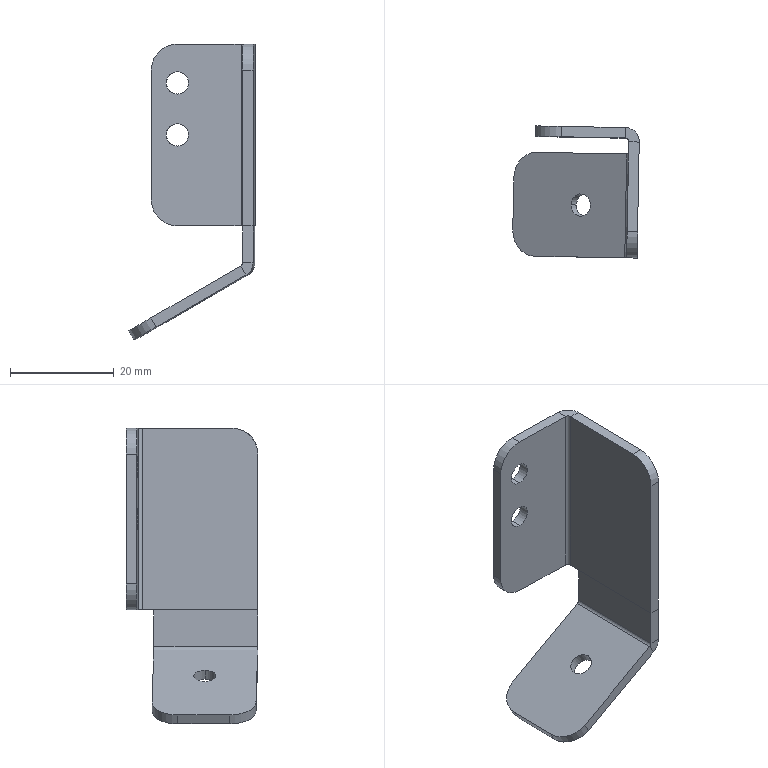Component | SolidWorks | DM17A08-02-004-1 | 2 solids | 39 faces | box 24.34 x 25.37 x 56.96 mm | volume 4173 mm3 | plane 24 | cylinder 15 | commonest cylinder face diameters 4.3 x6 10 x5 5.473 x2 1.473 x2
STEP:
#1=COLOUR_RGB('',0.7922,0.8196,0.9333);
#2=FILL_AREA_STYLE_COLOUR('',#1);
#3=FILL_AREA_STYLE('',(#2));
#4=SURFACE_STYLE_FILL_AREA(#3);
#5=SURFACE_SIDE_STYLE('',(#4));
#6=SURFACE_STYLE_USAGE(.BOTH.,#5);
#7=PRESENTATION_STYLE_ASSIGNMENT((#6));
#8=CARTESIAN_POINT('',(17.975,18.731,37.871));
#9=VERTEX_POINT('',#8);
#10=CARTESIAN_POINT('',(17.975,18.731,38.04));
#11=VERTEX_POINT('',#10);
#12=CARTESIAN_POINT('',(17.975,18.731,37.956));
#13=DIRECTION('',(0.01873,0.9998,-0.));
#14=DIRECTION('',(0.,0.,1.));
#15=AXIS2_PLACEMENT_3D('',#12,#13,#14);
#16=CIRCLE('',#15,0.08465);
#17=EDGE_CURVE('',#9,#11,#16,.T.);
#18=ORIENTED_EDGE('',*,*,#17,.F.);
#19=CARTESIAN_POINT('',(17.977,18.81,37.871));
#20=VERTEX_POINT('',#19);
#21=CARTESIAN_POINT('',(17.977,18.81,37.871));
#22=DIRECTION('',(0.01873,0.9998,-0.));
#23=VECTOR('',#22,39.37);
#24=LINE('',#21,#23);
#25=EDGE_CURVE('',#9,#20,#24,.T.);
#26=ORIENTED_EDGE('',*,*,#25,.T.);
#27=CARTESIAN_POINT('',(17.977,18.81,38.04));
#28=VERTEX_POINT('',#27);
#29=CARTESIAN_POINT('',(17.977,18.81,37.956));
#30=DIRECTION('',(0.01873,0.9998,-0.));
#31=DIRECTION('',(0.,0.,1.));
#32=AXIS2_PLACEMENT_3D('',#29,#30,#31);
#33=CIRCLE('',#32,0.08465);
#34=EDGE_CURVE('',#20,#28,#33,.T.);
#35=ORIENTED_EDGE('',*,*,#34,.T.);
#36=CARTESIAN_POINT('',(17.977,18.81,38.04));
#37=DIRECTION('',(0.01873,0.9998,-0.));
#38=VECTOR('',#37,39.37);
#39=LINE('',#36,#38);
#40=EDGE_CURVE('',#11,#28,#39,.T.);
#41=ORIENTED_EDGE('',*,*,#40,.F.);
#42=EDGE_LOOP('',(#18,#26,#35,#41));
#43=FACE_OUTER_BOUND('',#42,.T.);
#44=CARTESIAN_POINT('',(17.977,18.81,37.956));
#45=DIRECTION('',(0.01873,0.9998,-0.));
#46=DIRECTION('',(0.,0.,1.));
#47=AXIS2_PLACEMENT_3D('',#44,#45,#46);
#48=CYLINDRICAL_SURFACE('',#47,0.08465);
#49=ADVANCED_FACE('',(#43),#48,.F.);
#50=CARTESIAN_POINT('',(17.975,18.731,37.477));
#51=VERTEX_POINT('',#50);
#52=CARTESIAN_POINT('',(17.975,18.731,37.646));
#53=VERTEX_POINT('',#52);
#54=CARTESIAN_POINT('',(17.975,18.731,37.562));
#55=DIRECTION('',(0.01873,0.9998,-0.));
#56=DIRECTION('',(0.,0.,1.));
#57=AXIS2_PLACEMENT_3D('',#54,#55,#56);
#58=CIRCLE('',#57,0.08465);
#59=EDGE_CURVE('',#51,#53,#58,.T.);
#60=ORIENTED_EDGE('',*,*,#59,.F.);
#61=CARTESIAN_POINT('',(17.977,18.81,37.477));
#62=VERTEX_POINT('',#61);
#63=CARTESIAN_POINT('',(17.977,18.81,37.477));
#64=DIRECTION('',(0.01873,0.9998,-0.));
#65=VECTOR('',#64,39.37);
#66=LINE('',#63,#65);
#67=EDGE_CURVE('',#51,#62,#66,.T.);
#68=ORIENTED_EDGE('',*,*,#67,.T.);
#69=CARTESIAN_POINT('',(17.977,18.81,37.646));
#70=VERTEX_POINT('',#69);
#71=CARTESIAN_POINT('',(17.977,18.81,37.562));
#72=DIRECTION('',(0.01873,0.9998,-0.));
#73=DIRECTION('',(0.,0.,1.));
#74=AXIS2_PLACEMENT_3D('',#71,#72,#73);
#75=CIRCLE('',#74,0.08465);
#76=EDGE_CURVE('',#62,#70,#75,.T.);
#77=ORIENTED_EDGE('',*,*,#76,.T.);
#78=CARTESIAN_POINT('',(17.977,18.81,37.646));
#79=DIRECTION('',(0.01873,0.9998,-0.));
#80=VECTOR('',#79,39.37);
#81=LINE('',#78,#80);
#82=EDGE_CURVE('',#53,#70,#81,.T.);
#83=ORIENTED_EDGE('',*,*,#82,.F.);
#84=EDGE_LOOP('',(#60,#68,#77,#83));
#85=FACE_OUTER_BOUND('',#84,.T.);
#86=CARTESIAN_POINT('',(17.977,18.81,37.562));
#87=DIRECTION('',(0.01873,0.9998,-0.));
#88=DIRECTION('',(0.,0.,1.));
#89=AXIS2_PLACEMENT_3D('',#86,#87,#88);
#90=CYLINDRICAL_SURFACE('',#89,0.08465);
#91=ADVANCED_FACE('',(#85),#90,.F.);
#92=CARTESIAN_POINT('',(18.565,18.691,38.251));
#93=VERTEX_POINT('',#92);
#94=CARTESIAN_POINT('',(18.486,18.692,38.251));
#95=VERTEX_POINT('',#94);
#96=CARTESIAN_POINT('',(18.565,18.691,38.251));
#97=DIRECTION('',(-0.9998,0.01873,-0.));
#98=VECTOR('',#97,39.37);
#99=LINE('',#96,#98);
#100=EDGE_CURVE('',#93,#95,#99,.T.);
#101=ORIENTED_EDGE('',*,*,#100,.F.);
#102=CARTESIAN_POINT('',(18.459,18.801,38.251));
#103=VERTEX_POINT('',#102);
#104=CARTESIAN_POINT('',(18.457,18.693,38.251));
#105=DIRECTION('',(-0.,-0.,-1.));
#106=DIRECTION('',(0.9998,-0.01873,0.));
#107=AXIS2_PLACEMENT_3D('',#104,#105,#106);
#108=CIRCLE('',#107,0.1077);
#109=EDGE_CURVE('',#103,#93,#108,.T.);
#110=ORIENTED_EDGE('',*,*,#109,.F.);
#111=CARTESIAN_POINT('',(18.458,18.722,38.251));
#112=VERTEX_POINT('',#111);
#113=CARTESIAN_POINT('',(18.458,18.722,38.251));
#114=DIRECTION('',(0.01873,0.9998,-0.));
#115=VECTOR('',#114,39.37);
#116=LINE('',#113,#115);
#117=EDGE_CURVE('',#112,#103,#116,.T.);
#118=ORIENTED_EDGE('',*,*,#117,.F.);
#119=CARTESIAN_POINT('',(18.457,18.693,38.251));
#120=DIRECTION('',(-0.,-0.,-1.));
#121=DIRECTION('',(0.9998,-0.01873,0.));
#122=AXIS2_PLACEMENT_3D('',#119,#120,#121);
#123=CIRCLE('',#122,0.029);
#124=EDGE_CURVE('',#112,#95,#123,.T.);
#125=ORIENTED_EDGE('',*,*,#124,.T.);
#126=EDGE_LOOP('',(#101,#110,#118,#125));
#127=FACE_OUTER_BOUND('',#126,.T.);
#128=CARTESIAN_POINT('',(18.565,18.691,38.251));
#129=DIRECTION('',(0.,0.,1.));
#130=DIRECTION('',(0.9998,-0.01873,0.));
#131=AXIS2_PLACEMENT_3D('',#128,#129,#130);
#132=PLANE('',#131);
#133=ADVANCED_FACE('',(#127),#132,.T.);
#134=CARTESIAN_POINT('',(18.474,18.013,38.251));
#135=VERTEX_POINT('',#134);
#136=CARTESIAN_POINT('',(18.488,18.8,38.251));
#137=DIRECTION('',(-0.01873,-0.9998,0.));
#138=VECTOR('',#137,39.37);
#139=LINE('',#136,#138);
#140=EDGE_CURVE('',#95,#135,#139,.T.);
#141=ORIENTED_EDGE('',*,*,#140,.T.);
#142=CARTESIAN_POINT('',(18.552,18.011,38.251));
#143=VERTEX_POINT('',#142);
#144=CARTESIAN_POINT('',(18.445,18.013,38.251));
#145=DIRECTION('',(0.9998,-0.01873,0.));
#146=VECTOR('',#145,39.37);
#147=LINE('',#144,#146);
#148=EDGE_CURVE('',#135,#143,#147,.T.);
#149=ORIENTED_EDGE('',*,*,#148,.T.);
#150=CARTESIAN_POINT('',(18.567,18.799,38.251));
#151=DIRECTION('',(-0.01873,-0.9998,0.));
#152=VECTOR('',#151,39.37);
#153=LINE('',#150,#152);
#154=EDGE_CURVE('',#93,#143,#153,.T.);
#155=ORIENTED_EDGE('',*,*,#154,.F.);
#156=ORIENTED_EDGE('',*,*,#100,.T.);
#157=EDGE_LOOP('',(#141,#149,#155,#156));
#158=FACE_OUTER_BOUND('',#157,.T.);
#159=CARTESIAN_POINT('',(18.458,18.722,38.251));
#160=DIRECTION('',(0.,0.,1.));
#161=DIRECTION('',(0.9998,-0.01873,0.));
#162=AXIS2_PLACEMENT_3D('',#159,#160,#161);
#163=PLANE('',#162);
#164=ADVANCED_FACE('',(#158),#163,.T.);
#165=CARTESIAN_POINT('',(18.459,18.801,36.873));
#166=VERTEX_POINT('',#165);
#167=CARTESIAN_POINT('',(18.458,18.722,36.873));
#168=VERTEX_POINT('',#167);
#169=CARTESIAN_POINT('',(18.459,18.801,36.873));
#170=DIRECTION('',(-0.01873,-0.9998,0.));
#171=VECTOR('',#170,39.37);
#172=LINE('',#169,#171);
#173=EDGE_CURVE('',#166,#168,#172,.T.);
#174=ORIENTED_EDGE('',*,*,#173,.F.);
#175=CARTESIAN_POINT('',(18.565,18.691,36.873));
#176=VERTEX_POINT('',#175);
#177=CARTESIAN_POINT('',(18.457,18.693,36.873));
#178=DIRECTION('',(-0.,-0.,-1.));
#179=DIRECTION('',(0.9998,-0.01873,0.));
#180=AXIS2_PLACEMENT_3D('',#177,#178,#179);
#181=CIRCLE('',#180,0.1077);
#182=EDGE_CURVE('',#166,#176,#181,.T.);
#183=ORIENTED_EDGE('',*,*,#182,.T.);
#184=CARTESIAN_POINT('',(18.486,18.692,36.873));
#185=VERTEX_POINT('',#184);
#186=CARTESIAN_POINT('',(18.486,18.692,36.873));
#187=DIRECTION('',(0.9998,-0.01873,0.));
#188=VECTOR('',#187,39.37);
#189=LINE('',#186,#188);
#190=EDGE_CURVE('',#185,#176,#189,.T.);
#191=ORIENTED_EDGE('',*,*,#190,.F.);
#192=CARTESIAN_POINT('',(18.457,18.693,36.873));
#193=DIRECTION('',(-0.,-0.,-1.));
#194=DIRECTION('',(0.9998,-0.01873,0.));
#195=AXIS2_PLACEMENT_3D('',#192,#193,#194);
#196=CIRCLE('',#195,0.029);
#197=EDGE_CURVE('',#168,#185,#196,.T.);
#198=ORIENTED_EDGE('',*,*,#197,.F.);
#199=EDGE_LOOP('',(#174,#183,#191,#198));
#200=FACE_OUTER_BOUND('',#199,.T.);
#201=CARTESIAN_POINT('',(18.459,18.801,36.873));
#202=DIRECTION('',(-0.,-0.,-1.));
#203=DIRECTION('',(-0.9998,0.01873,-0.));
#204=AXIS2_PLACEMENT_3D('',#201,#202,#203);
#205=PLANE('',#204);
#206=ADVANCED_FACE('',(#200),#205,.T.);
#207=CARTESIAN_POINT('',(17.975,18.731,36.873));
#208=VERTEX_POINT('',#207);
#209=CARTESIAN_POINT('',(17.778,18.735,36.873));
#210=DIRECTION('',(0.9998,-0.01873,0.));
#211=VECTOR('',#210,39.37);
#212=LINE('',#209,#211);
#213=EDGE_CURVE('',#208,#168,#212,.T.);
#214=ORIENTED_EDGE('',*,*,#213,.F.);
#215=CARTESIAN_POINT('',(17.977,18.81,36.873));
#216=VERTEX_POINT('',#215);
#217=CARTESIAN_POINT('',(17.975,18.702,36.873));
#218=DIRECTION('',(0.01873,0.9998,-0.));
#219=VECTOR('',#218,39.37);
#220=LINE('',#217,#219);
#221=EDGE_CURVE('',#208,#216,#220,.T.);
#222=ORIENTED_EDGE('',*,*,#221,.T.);
#223=CARTESIAN_POINT('',(17.78,18.813,36.873));
#224=DIRECTION('',(0.9998,-0.01873,0.));
#225=VECTOR('',#224,39.37);
#226=LINE('',#223,#225);
#227=EDGE_CURVE('',#216,#166,#226,.T.);
#228=ORIENTED_EDGE('',*,*,#227,.T.);
#229=ORIENTED_EDGE('',*,*,#173,.T.);
#230=EDGE_LOOP('',(#214,#222,#228,#229));
#231=FACE_OUTER_BOUND('',#230,.T.);
#232=CARTESIAN_POINT('',(18.486,18.692,36.873));
#233=DIRECTION('',(-0.,-0.,-1.));
#234=DIRECTION('',(-0.9998,0.01873,-0.));
#235=AXIS2_PLACEMENT_3D('',#232,#233,#234);
#236=PLANE('',#235);
#237=ADVANCED_FACE('',(#231),#236,.T.);
#238=CARTESIAN_POINT('',(18.47,17.816,38.054));
#239=VERTEX_POINT('',#238);
#240=CARTESIAN_POINT('',(18.47,17.816,36.873));
#241=VERTEX_POINT('',#240);
#242=CARTESIAN_POINT('',(18.47,17.816,38.251));
#243=DIRECTION('',(-0.,-0.,-1.));
#244=VECTOR('',#243,39.37);
#245=LINE('',#242,#244);
#246=EDGE_CURVE('',#239,#241,#245,.T.);
#247=ORIENTED_EDGE('',*,*,#246,.F.);
#248=CARTESIAN_POINT('',(18.474,18.013,38.054));
#249=DIRECTION('',(-0.9998,0.01873,-0.));
#250=DIRECTION('',(0.01873,0.9998,0.));
#251=AXIS2_PLACEMENT_3D('',#248,#249,#250);
#252=CIRCLE('',#251,0.1969);
#253=EDGE_CURVE('',#239,#135,#252,.T.);
#254=ORIENTED_EDGE('',*,*,#253,.T.);
#255=ORIENTED_EDGE('',*,*,#140,.F.);
#256=CARTESIAN_POINT('',(18.486,18.692,38.251));
#257=DIRECTION('',(-0.,-0.,-1.));
#258=VECTOR('',#257,39.37);
#259=LINE('',#256,#258);
#260=EDGE_CURVE('',#95,#185,#259,.T.);
#261=ORIENTED_EDGE('',*,*,#260,.T.);
#262=CARTESIAN_POINT('',(18.488,18.8,36.873));
#263=DIRECTION('',(-0.01873,-0.9998,0.));
#264=VECTOR('',#263,39.37);
#265=LINE('',#262,#264);
#266=EDGE_CURVE('',#185,#241,#265,.T.);
#267=ORIENTED_EDGE('',*,*,#266,.T.);
#268=EDGE_LOOP('',(#247,#254,#255,#261,#267));
#269=FACE_OUTER_BOUND('',#268,.T.);
#270=CARTESIAN_POINT('',(18.488,18.8,38.251));
#271=DIRECTION('',(0.9998,-0.01873,0.));
#272=DIRECTION('',(0.01873,0.9998,-0.));
#273=AXIS2_PLACEMENT_3D('',#270,#271,#272);
#274=PLANE('',#273);
#275=ADVANCED_FACE('',(#269),#274,.F.);
#276=CARTESIAN_POINT('',(18.549,17.815,38.054));
#277=VERTEX_POINT('',#276);
#278=CARTESIAN_POINT('',(18.549,17.815,36.873));
#279=VERTEX_POINT('',#278);
#280=CARTESIAN_POINT('',(18.549,17.815,38.251));
#281=DIRECTION('',(-0.,-0.,-1.));
#282=VECTOR('',#281,39.37);
#283=LINE('',#280,#282);
#284=EDGE_CURVE('',#277,#279,#283,.T.);
#285=ORIENTED_EDGE('',*,*,#284,.F.);
#286=CARTESIAN_POINT('',(18.549,17.815,38.054));
#287=DIRECTION('',(-0.9998,0.01873,-0.));
#288=VECTOR('',#287,39.37);
#289=LINE('',#286,#288);
#290=EDGE_CURVE('',#277,#239,#289,.T.);
#291=ORIENTED_EDGE('',*,*,#290,.T.);
#292=ORIENTED_EDGE('',*,*,#246,.T.);
#293=CARTESIAN_POINT('',(18.549,17.815,36.873));
#294=DIRECTION('',(-0.9998,0.01873,-0.));
#295=VECTOR('',#294,39.37);
#296=LINE('',#293,#295);
#297=EDGE_CURVE('',#279,#241,#296,.T.);
#298=ORIENTED_EDGE('',*,*,#297,.F.);
#299=EDGE_LOOP('',(#285,#291,#292,#298));
#300=FACE_OUTER_BOUND('',#299,.T.);
#301=CARTESIAN_POINT('',(18.549,17.815,38.251));
#302=DIRECTION('',(-0.01873,-0.9998,0.));
#303=DIRECTION('',(-0.,-0.,-1.));
#304=AXIS2_PLACEMENT_3D('',#301,#302,#303);
#305=PLANE('',#304);
#306=ADVANCED_FACE('',(#300),#305,.T.);
#307=ORIENTED_EDGE('',*,*,#154,.T.);
#308=CARTESIAN_POINT('',(18.552,18.011,38.054));
#309=DIRECTION('',(0.9998,-0.01873,0.));
#310=DIRECTION('',(0.01873,0.9998,0.));
#311=AXIS2_PLACEMENT_3D('',#308,#309,#310);
#312=CIRCLE('',#311,0.1969);
#313=EDGE_CURVE('',#143,#277,#312,.T.);
#314=ORIENTED_EDGE('',*,*,#313,.T.);
#315=ORIENTED_EDGE('',*,*,#284,.T.);
#316=CARTESIAN_POINT('',(18.567,18.799,36.873));
#317=DIRECTION('',(-0.01873,-0.9998,0.));
#318=VECTOR('',#317,39.37);
#319=LINE('',#316,#318);
#320=EDGE_CURVE('',#176,#279,#319,.T.);
#321=ORIENTED_EDGE('',*,*,#320,.F.);
#322=CARTESIAN_POINT('',(18.565,18.691,38.251));
#323=DIRECTION('',(-0.,-0.,-1.));
#324=VECTOR('',#323,39.37);
#325=LINE('',#322,#324);
#326=EDGE_CURVE('',#93,#176,#325,.T.);
#327=ORIENTED_EDGE('',*,*,#326,.F.);
#328=EDGE_LOOP('',(#307,#314,#315,#321,#327));
#329=FACE_OUTER_BOUND('',#328,.T.);
#330=CARTESIAN_POINT('',(18.567,18.799,38.251));
#331=DIRECTION('',(0.9998,-0.01873,0.));
#332=DIRECTION('',(0.01873,0.9998,-0.));
#333=AXIS2_PLACEMENT_3D('',#330,#331,#332);
#334=PLANE('',#333);
#335=ADVANCED_FACE('',(#329),#334,.T.);
#336=ORIENTED_EDGE('',*,*,#182,.F.);
#337=CARTESIAN_POINT('',(18.459,18.801,38.251));
#338=DIRECTION('',(-0.,-0.,-1.));
#339=VECTOR('',#338,39.37);
#340=LINE('',#337,#339);
#341=EDGE_CURVE('',#103,#166,#340,.T.);
#342=ORIENTED_EDGE('',*,*,#341,.F.);
#343=ORIENTED_EDGE('',*,*,#109,.T.);
#344=ORIENTED_EDGE('',*,*,#326,.T.);
#345=EDGE_LOOP('',(#336,#342,#343,#344));
#346=FACE_OUTER_BOUND('',#345,.T.);
#347=CARTESIAN_POINT('',(18.457,18.693,38.251));
#348=DIRECTION('',(-0.,-0.,-1.));
#349=DIRECTION('',(-0.9998,0.01873,0.));
#350=AXIS2_PLACEMENT_3D('',#347,#348,#349);
#351=CYLINDRICAL_SURFACE('',#350,0.1077);
#352=ADVANCED_FACE('',(#346),#351,.T.);
#353=CARTESIAN_POINT('',(17.977,18.81,37.956));
#354=DIRECTION('',(0.01873,0.9998,-0.));
#355=DIRECTION('',(0.,0.,1.));
#356=AXIS2_PLACEMENT_3D('',#353,#354,#355);
#357=CIRCLE('',#356,0.08465);
#358=EDGE_CURVE('',#28,#20,#357,.T.);
#359=ORIENTED_EDGE('',*,*,#358,.F.);
#360=ORIENTED_EDGE('',*,*,#34,.F.);
#361=EDGE_LOOP('',(#359,#360));
#362=FACE_BOUND('',#361,.T.);
#363=CARTESIAN_POINT('',(17.977,18.81,37.562));
#364=DIRECTION('',(0.01873,0.9998,-0.));
#365=DIRECTION('',(0.,0.,1.));
#366=AXIS2_PLACEMENT_3D('',#363,#364,#365);
#367=CIRCLE('',#366,0.08465);
#368=EDGE_CURVE('',#70,#62,#367,.T.);
#369=ORIENTED_EDGE('',*,*,#368,.F.);
#370=ORIENTED_EDGE('',*,*,#76,.F.);
#371=EDGE_LOOP('',(#369,#370));
#372=FACE_BOUND('',#371,.T.);
#373=ORIENTED_EDGE('',*,*,#227,.F.);
#374=CARTESIAN_POINT('',(17.78,18.813,37.069));
#375=VERTEX_POINT('',#374);
#376=CARTESIAN_POINT('',(17.977,18.81,37.069));
#377=DIRECTION('',(0.01873,0.9998,-0.));
#378=DIRECTION('',(0.,0.,1.));
#379=AXIS2_PLACEMENT_3D('',#376,#377,#378);
#380=CIRCLE('',#379,0.1969);
#381=EDGE_CURVE('',#216,#375,#380,.T.);
#382=ORIENTED_EDGE('',*,*,#381,.T.);
#383=CARTESIAN_POINT('',(17.78,18.813,38.054));
#384=VERTEX_POINT('',#383);
#385=CARTESIAN_POINT('',(17.78,18.813,38.251));
#386=DIRECTION('',(-0.,-0.,-1.));
#387=VECTOR('',#386,39.37);
#388=LINE('',#385,#387);
#389=EDGE_CURVE('',#384,#375,#388,.T.);
#390=ORIENTED_EDGE('',*,*,#389,.F.);
#391=CARTESIAN_POINT('',(17.977,18.81,38.251));
#392=VERTEX_POINT('',#391);
#393=CARTESIAN_POINT('',(17.977,18.81,38.054));
#394=DIRECTION('',(0.01873,0.9998,-0.));
#395=DIRECTION('',(0.,0.,1.));
#396=AXIS2_PLACEMENT_3D('',#393,#394,#395);
#397=CIRCLE('',#396,0.1969);
#398=EDGE_CURVE('',#384,#392,#397,.T.);
#399=ORIENTED_EDGE('',*,*,#398,.T.);
#400=CARTESIAN_POINT('',(17.78,18.813,38.251));
#401=DIRECTION('',(0.9998,-0.01873,0.));
#402=VECTOR('',#401,39.37);
#403=LINE('',#400,#402);
#404=EDGE_CURVE('',#392,#103,#403,.T.);
#405=ORIENTED_EDGE('',*,*,#404,.T.);
#406=ORIENTED_EDGE('',*,*,#341,.T.);
#407=EDGE_LOOP('',(#373,#382,#390,#399,#405,#406));
#408=FACE_OUTER_BOUND('',#407,.T.);
#409=CARTESIAN_POINT('',(17.78,18.813,38.251));
#410=DIRECTION('',(0.01873,0.9998,-0.));
#411=DIRECTION('',(0.,0.,1.));
#412=AXIS2_PLACEMENT_3D('',#409,#410,#411);
#413=PLANE('',#412);
#414=ADVANCED_FACE('',(#362,#372,#408),#413,.T.);
#415=ORIENTED_EDGE('',*,*,#389,.T.);
#416=CARTESIAN_POINT('',(17.778,18.735,37.069));
#417=VERTEX_POINT('',#416);
#418=CARTESIAN_POINT('',(17.778,18.735,37.069));
#419=DIRECTION('',(-0.01873,-0.9998,0.));
#420=VECTOR('',#419,39.37);
#421=LINE('',#418,#420);
#422=EDGE_CURVE('',#375,#417,#421,.T.);
#423=ORIENTED_EDGE('',*,*,#422,.T.);
#424=CARTESIAN_POINT('',(17.778,18.735,38.054));
#425=VERTEX_POINT('',#424);
#426=CARTESIAN_POINT('',(17.778,18.735,38.251));
#427=DIRECTION('',(-0.,-0.,-1.));
#428=VECTOR('',#427,39.37);
#429=LINE('',#426,#428);
#430=EDGE_CURVE('',#425,#417,#429,.T.);
#431=ORIENTED_EDGE('',*,*,#430,.F.);
#432=CARTESIAN_POINT('',(17.778,18.735,38.054));
#433=DIRECTION('',(0.01873,0.9998,-0.));
#434=VECTOR('',#433,39.37);
#435=LINE('',#432,#434);
#436=EDGE_CURVE('',#425,#384,#435,.T.);
#437=ORIENTED_EDGE('',*,*,#436,.T.);
#438=EDGE_LOOP('',(#415,#423,#431,#437));
#439=FACE_OUTER_BOUND('',#438,.T.);
#440=CARTESIAN_POINT('',(17.778,18.735,38.251));
#441=DIRECTION('',(-0.9998,0.01873,-0.));
#442=DIRECTION('',(0.,0.,1.));
#443=AXIS2_PLACEMENT_3D('',#440,#441,#442);
#444=PLANE('',#443);
#445=ADVANCED_FACE('',(#439),#444,.T.);
#446=CARTESIAN_POINT('',(17.975,18.731,37.956));
#447=DIRECTION('',(0.01873,0.9998,-0.));
#448=DIRECTION('',(0.,0.,1.));
#449=AXIS2_PLACEMENT_3D('',#446,#447,#448);
#450=CIRCLE('',#449,0.08465);
#451=EDGE_CURVE('',#11,#9,#450,.T.);
#452=ORIENTED_EDGE('',*,*,#451,.T.);
#453=ORIENTED_EDGE('',*,*,#17,.T.);
#454=EDGE_LOOP('',(#452,#453));
#455=FACE_BOUND('',#454,.T.);
#456=CARTESIAN_POINT('',(17.975,18.731,37.562));
#457=DIRECTION('',(0.01873,0.9998,-0.));
#458=DIRECTION('',(0.,0.,1.));
#459=AXIS2_PLACEMENT_3D('',#456,#457,#458);
#460=CIRCLE('',#459,0.08465);
#461=EDGE_CURVE('',#53,#51,#460,.T.);
#462=ORIENTED_EDGE('',*,*,#461,.T.);
#463=ORIENTED_EDGE('',*,*,#59,.T.);
#464=EDGE_LOOP('',(#462,#463));
#465=FACE_BOUND('',#464,.T.);
#466=ORIENTED_EDGE('',*,*,#430,.T.);
#467=CARTESIAN_POINT('',(17.975,18.731,37.069));
#468=DIRECTION('',(-0.01873,-0.9998,0.));
#469=DIRECTION('',(0.,0.,1.));
#470=AXIS2_PLACEMENT_3D('',#467,#468,#469);
#471=CIRCLE('',#470,0.1969);
#472=EDGE_CURVE('',#417,#208,#471,.T.);
#473=ORIENTED_EDGE('',*,*,#472,.T.);
#474=ORIENTED_EDGE('',*,*,#213,.T.);
#475=CARTESIAN_POINT('',(18.458,18.722,38.251));
#476=DIRECTION('',(-0.,-0.,-1.));
#477=VECTOR('',#476,39.37);
#478=LINE('',#475,#477);
#479=EDGE_CURVE('',#112,#168,#478,.T.);
#480=ORIENTED_EDGE('',*,*,#479,.F.);
#481=CARTESIAN_POINT('',(17.975,18.731,38.251));
#482=VERTEX_POINT('',#481);
#483=CARTESIAN_POINT('',(17.778,18.735,38.251));
#484=DIRECTION('',(0.9998,-0.01873,0.));
#485=VECTOR('',#484,39.37);
#486=LINE('',#483,#485);
#487=EDGE_CURVE('',#482,#112,#486,.T.);
#488=ORIENTED_EDGE('',*,*,#487,.F.);
#489=CARTESIAN_POINT('',(17.975,18.731,38.054));
#490=DIRECTION('',(-0.01873,-0.9998,0.));
#491=DIRECTION('',(0.,0.,1.));
#492=AXIS2_PLACEMENT_3D('',#489,#490,#491);
#493=CIRCLE('',#492,0.1969);
#494=EDGE_CURVE('',#482,#425,#493,.T.);
#495=ORIENTED_EDGE('',*,*,#494,.T.);
#496=EDGE_LOOP('',(#466,#473,#474,#480,#488,#495));
#497=FACE_OUTER_BOUND('',#496,.T.);
#498=CARTESIAN_POINT('',(17.778,18.735,38.251));
#499=DIRECTION('',(0.01873,0.9998,-0.));
#500=DIRECTION('',(0.,0.,1.));
#501=AXIS2_PLACEMENT_3D('',#498,#499,#500);
#502=PLANE('',#501);
#503=ADVANCED_FACE('',(#455,#465,#497),#502,.F.);
#504=ORIENTED_EDGE('',*,*,#197,.T.);
#505=ORIENTED_EDGE('',*,*,#260,.F.);
#506=ORIENTED_EDGE('',*,*,#124,.F.);
#507=ORIENTED_EDGE('',*,*,#479,.T.);
#508=EDGE_LOOP('',(#504,#505,#506,#507));
#509=FACE_OUTER_BOUND('',#508,.T.);
#510=CARTESIAN_POINT('',(18.457,18.693,38.251));
#511=DIRECTION('',(-0.,-0.,-1.));
#512=DIRECTION('',(-0.9998,0.01873,0.));
#513=AXIS2_PLACEMENT_3D('',#510,#511,#512);
#514=CYLINDRICAL_SURFACE('',#513,0.029);
#515=ADVANCED_FACE('',(#509),#514,.F.);
#516=ORIENTED_EDGE('',*,*,#404,.F.);
#517=CARTESIAN_POINT('',(17.975,18.702,38.251));
#518=DIRECTION('',(-0.01873,-0.9998,0.));
#519=VECTOR('',#518,39.37);
#520=LINE('',#517,#519);
#521=EDGE_CURVE('',#392,#482,#520,.T.);
#522=ORIENTED_EDGE('',*,*,#521,.T.);
#523=ORIENTED_EDGE('',*,*,#487,.T.);
#524=ORIENTED_EDGE('',*,*,#117,.T.);
#525=EDGE_LOOP('',(#516,#522,#523,#524));
#526=FACE_OUTER_BOUND('',#525,.T.);
#527=CARTESIAN_POINT('',(18.457,18.693,38.251));
#528=DIRECTION('',(0.,0.,1.));
#529=DIRECTION('',(0.9998,-0.01873,0.));
#530=AXIS2_PLACEMENT_3D('',#527,#528,#529);
#531=PLANE('',#530);
#532=ADVANCED_FACE('',(#526),#531,.T.);
#533=ORIENTED_EDGE('',*,*,#266,.F.);
#534=ORIENTED_EDGE('',*,*,#190,.T.);
#535=ORIENTED_EDGE('',*,*,#320,.T.);
#536=ORIENTED_EDGE('',*,*,#297,.T.);
#537=EDGE_LOOP('',(#533,#534,#535,#536));
#538=FACE_OUTER_BOUND('',#537,.T.);
#539=CARTESIAN_POINT('',(18.457,18.693,36.873));
#540=DIRECTION('',(0.,0.,1.));
#541=DIRECTION('',(0.9998,-0.01873,0.));
#542=AXIS2_PLACEMENT_3D('',#539,#540,#541);
#543=PLANE('',#542);
#544=ADVANCED_FACE('',(#538),#543,.F.);
#545=ORIENTED_EDGE('',*,*,#67,.F.);
#546=ORIENTED_EDGE('',*,*,#461,.F.);
#547=ORIENTED_EDGE('',*,*,#82,.T.);
#548=ORIENTED_EDGE('',*,*,#368,.T.);
#549=EDGE_LOOP('',(#545,#546,#547,#548));
#550=FACE_OUTER_BOUND('',#549,.T.);
#551=CARTESIAN_POINT('',(17.977,18.81,37.562));
#552=DIRECTION('',(0.01873,0.9998,-0.));
#553=DIRECTION('',(0.,0.,1.));
#554=AXIS2_PLACEMENT_3D('',#551,#552,#553);
#555=CYLINDRICAL_SURFACE('',#554,0.08465);
#556=ADVANCED_FACE('',(#550),#555,.F.);
#557=ORIENTED_EDGE('',*,*,#25,.F.);
#558=ORIENTED_EDGE('',*,*,#451,.F.);
#559=ORIENTED_EDGE('',*,*,#40,.T.);
#560=ORIENTED_EDGE('',*,*,#358,.T.);
#561=EDGE_LOOP('',(#557,#558,#559,#560));
#562=FACE_OUTER_BOUND('',#561,.T.);
#563=CARTESIAN_POINT('',(17.977,18.81,37.956));
#564=DIRECTION('',(0.01873,0.9998,-0.));
#565=DIRECTION('',(0.,0.,1.));
#566=AXIS2_PLACEMENT_3D('',#563,#564,#565);
#567=CYLINDRICAL_SURFACE('',#566,0.08465);
#568=ADVANCED_FACE('',(#562),#567,.F.);
#569=ORIENTED_EDGE('',*,*,#472,.F.);
#570=ORIENTED_EDGE('',*,*,#422,.F.);
#571=ORIENTED_EDGE('',*,*,#381,.F.);
#572=ORIENTED_EDGE('',*,*,#221,.F.);
#573=EDGE_LOOP('',(#569,#570,#571,#572));
#574=FACE_OUTER_BOUND('',#573,.T.);
#575=CARTESIAN_POINT('',(17.975,18.702,37.069));
#576=DIRECTION('',(0.01873,0.9998,-0.));
#577=DIRECTION('',(0.,0.,1.));
#578=AXIS2_PLACEMENT_3D('',#575,#576,#577);
#579=CYLINDRICAL_SURFACE('',#578,0.1969);
#580=ADVANCED_FACE('',(#574),#579,.T.);
#581=ORIENTED_EDGE('',*,*,#313,.F.);
#582=ORIENTED_EDGE('',*,*,#148,.F.);
#583=ORIENTED_EDGE('',*,*,#253,.F.);
#584=ORIENTED_EDGE('',*,*,#290,.F.);
#585=EDGE_LOOP('',(#581,#582,#583,#584));
#586=FACE_OUTER_BOUND('',#585,.T.);
#587=CARTESIAN_POINT('',(18.552,18.011,38.054));
#588=DIRECTION('',(-0.9998,0.01873,-0.));
#589=DIRECTION('',(0.,0.,1.));
#590=AXIS2_PLACEMENT_3D('',#587,#588,#589);
#591=CYLINDRICAL_SURFACE('',#590,0.1969);
#592=ADVANCED_FACE('',(#586),#591,.T.);
#593=ORIENTED_EDGE('',*,*,#494,.F.);
#594=ORIENTED_EDGE('',*,*,#521,.F.);
#595=ORIENTED_EDGE('',*,*,#398,.F.);
#596=ORIENTED_EDGE('',*,*,#436,.F.);
#597=EDGE_LOOP('',(#593,#594,#595,#596));
#598=FACE_OUTER_BOUND('',#597,.T.);
#599=CARTESIAN_POINT('',(17.975,18.731,38.054));
#600=DIRECTION('',(0.01873,0.9998,-0.));
#601=DIRECTION('',(0.,0.,1.));
#602=AXIS2_PLACEMENT_3D('',#599,#600,#601);
#603=CYLINDRICAL_SURFACE('',#602,0.1969);
#604=ADVANCED_FACE('',(#598),#603,.T.);
#605=CLOSED_SHELL('',(#49,#91,#133,#164,#206,#237,#275,#306,#335,#352,#414,#445,#503,#515,#532,#544,#556,#568,#580,#592,#604));
#606=MANIFOLD_SOLID_BREP('',#605);
#607=STYLED_ITEM('',(#7),#606);
#608=PRESENTATION_LAYER_ASSIGNMENT('','',(#607));
#609=COLOUR_RGB('',0.7922,0.8196,0.9333);
#610=FILL_AREA_STYLE_COLOUR('',#609);
#611=FILL_AREA_STYLE('',(#610));
#612=SURFACE_STYLE_FILL_AREA(#611);
#613=SURFACE_SIDE_STYLE('',(#612));
#614=SURFACE_STYLE_USAGE(.BOTH.,#613);
#615=PRESENTATION_STYLE_ASSIGNMENT((#614));
#616=CARTESIAN_POINT('',(18.088,18.217,36.261));
#617=VERTEX_POINT('',#616);
#618=CARTESIAN_POINT('',(18.235,18.214,36.346));
#619=VERTEX_POINT('',#618);
#620=CARTESIAN_POINT('',(18.161,18.216,36.303));
#621=DIRECTION('',(-0.4999,0.009366,0.866));
#622=DIRECTION('',(0.8659,-0.01622,0.5));
#623=AXIS2_PLACEMENT_3D('',#620,#621,#622);
#624=CIRCLE('',#623,0.08465);
#625=EDGE_CURVE('',#617,#619,#624,.T.);
#626=ORIENTED_EDGE('',*,*,#625,.F.);
#627=CARTESIAN_POINT('',(18.049,18.218,36.329));
#628=VERTEX_POINT('',#627);
#629=CARTESIAN_POINT('',(18.049,18.218,36.329));
#630=DIRECTION('',(-0.4999,0.009366,0.866));
#631=VECTOR('',#630,39.37);
#632=LINE('',#629,#631);
#633=EDGE_CURVE('',#617,#628,#632,.T.);
#634=ORIENTED_EDGE('',*,*,#633,.T.);
#635=CARTESIAN_POINT('',(18.195,18.215,36.414));
#636=VERTEX_POINT('',#635);
#637=CARTESIAN_POINT('',(18.122,18.216,36.371));
#638=DIRECTION('',(-0.4999,0.009366,0.866));
#639=DIRECTION('',(0.8659,-0.01622,0.5));
#640=AXIS2_PLACEMENT_3D('',#637,#638,#639);
#641=CIRCLE('',#640,0.08465);
#642=EDGE_CURVE('',#628,#636,#641,.T.);
#643=ORIENTED_EDGE('',*,*,#642,.T.);
#644=CARTESIAN_POINT('',(18.195,18.215,36.414));
#645=DIRECTION('',(-0.4999,0.009366,0.866));
#646=VECTOR('',#645,39.37);
#647=LINE('',#644,#646);
#648=EDGE_CURVE('',#619,#636,#647,.T.);
#649=ORIENTED_EDGE('',*,*,#648,.F.);
#650=EDGE_LOOP('',(#626,#634,#643,#649));
#651=FACE_OUTER_BOUND('',#650,.T.);
#652=CARTESIAN_POINT('',(18.122,18.216,36.371));
#653=DIRECTION('',(-0.4999,0.009366,0.866));
#654=DIRECTION('',(0.8659,-0.01622,0.5));
#655=AXIS2_PLACEMENT_3D('',#652,#653,#654);
#656=CYLINDRICAL_SURFACE('',#655,0.08465);
#657=ADVANCED_FACE('',(#651),#656,.F.);
#658=CARTESIAN_POINT('',(18.161,18.216,36.303));
#659=DIRECTION('',(-0.4999,0.009366,0.866));
#660=DIRECTION('',(0.8659,-0.01622,0.5));
#661=AXIS2_PLACEMENT_3D('',#658,#659,#660);
#662=CIRCLE('',#661,0.08465);
#663=EDGE_CURVE('',#619,#617,#662,.T.);
#664=ORIENTED_EDGE('',*,*,#663,.T.);
#665=ORIENTED_EDGE('',*,*,#625,.T.);
#666=EDGE_LOOP('',(#664,#665));
#667=FACE_BOUND('',#666,.T.);
#668=CARTESIAN_POINT('',(17.646,18.028,36.008));
#669=VERTEX_POINT('',#668);
#670=CARTESIAN_POINT('',(17.654,18.422,36.008));
#671=VERTEX_POINT('',#670);
#672=CARTESIAN_POINT('',(17.657,18.619,36.008));
#673=DIRECTION('',(0.01873,0.9998,-0.));
#674=VECTOR('',#673,39.37);
#675=LINE('',#672,#674);
#676=EDGE_CURVE('',#669,#671,#675,.T.);
#677=ORIENTED_EDGE('',*,*,#676,.T.);
#678=CARTESIAN_POINT('',(17.828,18.616,36.106));
#679=VERTEX_POINT('',#678);
#680=CARTESIAN_POINT('',(17.824,18.419,36.106));
#681=DIRECTION('',(0.4999,-0.009366,-0.866));
#682=DIRECTION('',(0.8659,-0.01622,0.5));
#683=AXIS2_PLACEMENT_3D('',#680,#681,#682);
#684=CIRCLE('',#683,0.1969);
#685=EDGE_CURVE('',#671,#679,#684,.T.);
#686=ORIENTED_EDGE('',*,*,#685,.T.);
#687=CARTESIAN_POINT('',(18.509,18.603,36.5));
#688=VERTEX_POINT('',#687);
#689=CARTESIAN_POINT('',(18.813,18.597,36.675));
#690=DIRECTION('',(-0.8659,0.01622,-0.5));
#691=VECTOR('',#690,39.37);
#692=LINE('',#689,#691);
#693=EDGE_CURVE('',#688,#679,#692,.T.);
#694=ORIENTED_EDGE('',*,*,#693,.F.);
#695=CARTESIAN_POINT('',(18.495,17.816,36.5));
#696=VERTEX_POINT('',#695);
#697=CARTESIAN_POINT('',(18.509,18.603,36.5));
#698=DIRECTION('',(0.01873,0.9998,-0.));
#699=VECTOR('',#698,39.37);
#700=LINE('',#697,#699);
#701=EDGE_CURVE('',#696,#688,#700,.T.);
#702=ORIENTED_EDGE('',*,*,#701,.F.);
#703=CARTESIAN_POINT('',(17.813,17.828,36.106));
#704=VERTEX_POINT('',#703);
#705=CARTESIAN_POINT('',(18.798,17.81,36.675));
#706=DIRECTION('',(-0.8659,0.01622,-0.5));
#707=VECTOR('',#706,39.37);
#708=LINE('',#705,#707);
#709=EDGE_CURVE('',#696,#704,#708,.T.);
#710=ORIENTED_EDGE('',*,*,#709,.T.);
#711=CARTESIAN_POINT('',(17.817,18.025,36.106));
#712=DIRECTION('',(0.4999,-0.009366,-0.866));
#713=DIRECTION('',(0.8659,-0.01622,0.5));
#714=AXIS2_PLACEMENT_3D('',#711,#712,#713);
#715=CIRCLE('',#714,0.1969);
#716=EDGE_CURVE('',#704,#669,#715,.T.);
#717=ORIENTED_EDGE('',*,*,#716,.T.);
#718=EDGE_LOOP('',(#677,#686,#694,#702,#710,#717));
#719=FACE_OUTER_BOUND('',#718,.T.);
#720=CARTESIAN_POINT('',(18.813,18.597,36.675));
#721=DIRECTION('',(-0.4999,0.009366,0.866));
#722=DIRECTION('',(0.8659,-0.01622,0.5));
#723=AXIS2_PLACEMENT_3D('',#720,#721,#722);
#724=PLANE('',#723);
#725=ADVANCED_FACE('',(#667,#719),#724,.F.);
#726=CARTESIAN_POINT('',(18.455,17.816,36.568));
#727=VERTEX_POINT('',#726);
#728=CARTESIAN_POINT('',(17.774,17.829,36.175));
#729=VERTEX_POINT('',#728);
#730=CARTESIAN_POINT('',(18.759,17.811,36.744));
#731=DIRECTION('',(-0.8659,0.01622,-0.5));
#732=VECTOR('',#731,39.37);
#733=LINE('',#730,#732);
#734=EDGE_CURVE('',#727,#729,#733,.T.);
#735=ORIENTED_EDGE('',*,*,#734,.T.);
#736=CARTESIAN_POINT('',(17.813,17.828,36.106));
#737=DIRECTION('',(0.4999,-0.009366,-0.866));
#738=VECTOR('',#737,39.37);
#739=LINE('',#736,#738);
#740=EDGE_CURVE('',#729,#704,#739,.T.);
#741=ORIENTED_EDGE('',*,*,#740,.T.);
#742=ORIENTED_EDGE('',*,*,#709,.F.);
#743=CARTESIAN_POINT('',(18.495,17.816,36.5));
#744=DIRECTION('',(0.4999,-0.009366,-0.866));
#745=VECTOR('',#744,39.37);
#746=LINE('',#743,#745);
#747=EDGE_CURVE('',#727,#696,#746,.T.);
#748=ORIENTED_EDGE('',*,*,#747,.F.);
#749=EDGE_LOOP('',(#735,#741,#742,#748));
#750=FACE_OUTER_BOUND('',#749,.T.);
#751=CARTESIAN_POINT('',(18.798,17.81,36.675));
#752=DIRECTION('',(0.01873,0.9998,-0.));
#753=DIRECTION('',(-0.4999,0.009366,0.866));
#754=AXIS2_PLACEMENT_3D('',#751,#752,#753);
#755=PLANE('',#754);
#756=ADVANCED_FACE('',(#750),#755,.F.);
#757=ORIENTED_EDGE('',*,*,#693,.T.);
#758=CARTESIAN_POINT('',(17.788,18.616,36.175));
#759=VERTEX_POINT('',#758);
#760=CARTESIAN_POINT('',(17.788,18.616,36.175));
#761=DIRECTION('',(-0.4999,0.009366,0.866));
#762=VECTOR('',#761,39.37);
#763=LINE('',#760,#762);
#764=EDGE_CURVE('',#679,#759,#763,.T.);
#765=ORIENTED_EDGE('',*,*,#764,.T.);
#766=CARTESIAN_POINT('',(18.47,18.604,36.568));
#767=VERTEX_POINT('',#766);
#768=CARTESIAN_POINT('',(18.774,18.598,36.744));
#769=DIRECTION('',(-0.8659,0.01622,-0.5));
#770=VECTOR('',#769,39.37);
#771=LINE('',#768,#770);
#772=EDGE_CURVE('',#767,#759,#771,.T.);
#773=ORIENTED_EDGE('',*,*,#772,.F.);
#774=CARTESIAN_POINT('',(18.509,18.603,36.5));
#775=DIRECTION('',(0.4999,-0.009366,-0.866));
#776=VECTOR('',#775,39.37);
#777=LINE('',#774,#776);
#778=EDGE_CURVE('',#767,#688,#777,.T.);
#779=ORIENTED_EDGE('',*,*,#778,.T.);
#780=EDGE_LOOP('',(#757,#765,#773,#779));
#781=FACE_OUTER_BOUND('',#780,.T.);
#782=CARTESIAN_POINT('',(18.813,18.597,36.675));
#783=DIRECTION('',(0.01873,0.9998,-0.));
#784=DIRECTION('',(-0.4999,0.009366,0.866));
#785=AXIS2_PLACEMENT_3D('',#782,#783,#784);
#786=PLANE('',#785);
#787=ADVANCED_FACE('',(#781),#786,.T.);
#788=CARTESIAN_POINT('',(18.122,18.216,36.371));
#789=DIRECTION('',(-0.4999,0.009366,0.866));
#790=DIRECTION('',(0.8659,-0.01622,0.5));
#791=AXIS2_PLACEMENT_3D('',#788,#789,#790);
#792=CIRCLE('',#791,0.08465);
#793=EDGE_CURVE('',#636,#628,#792,.T.);
#794=ORIENTED_EDGE('',*,*,#793,.F.);
#795=ORIENTED_EDGE('',*,*,#642,.F.);
#796=EDGE_LOOP('',(#794,#795));
#797=FACE_BOUND('',#796,.T.);
#798=ORIENTED_EDGE('',*,*,#772,.T.);
#799=CARTESIAN_POINT('',(17.614,18.423,36.076));
#800=VERTEX_POINT('',#799);
#801=CARTESIAN_POINT('',(17.785,18.42,36.175));
#802=DIRECTION('',(-0.4999,0.009366,0.866));
#803=DIRECTION('',(0.8659,-0.01622,0.5));
#804=AXIS2_PLACEMENT_3D('',#801,#802,#803);
#805=CIRCLE('',#804,0.1969);
#806=EDGE_CURVE('',#759,#800,#805,.T.);
#807=ORIENTED_EDGE('',*,*,#806,.T.);
#808=CARTESIAN_POINT('',(17.607,18.029,36.076));
#809=VERTEX_POINT('',#808);
#810=CARTESIAN_POINT('',(17.618,18.62,36.076));
#811=DIRECTION('',(0.01873,0.9998,-0.));
#812=VECTOR('',#811,39.37);
#813=LINE('',#810,#812);
#814=EDGE_CURVE('',#809,#800,#813,.T.);
#815=ORIENTED_EDGE('',*,*,#814,.F.);
#816=CARTESIAN_POINT('',(17.777,18.026,36.175));
#817=DIRECTION('',(-0.4999,0.009366,0.866));
#818=DIRECTION('',(0.8659,-0.01622,0.5));
#819=AXIS2_PLACEMENT_3D('',#816,#817,#818);
#820=CIRCLE('',#819,0.1969);
#821=EDGE_CURVE('',#809,#729,#820,.T.);
#822=ORIENTED_EDGE('',*,*,#821,.T.);
#823=ORIENTED_EDGE('',*,*,#734,.F.);
#824=CARTESIAN_POINT('',(18.47,18.604,36.568));
#825=DIRECTION('',(0.01873,0.9998,-0.));
#826=VECTOR('',#825,39.37);
#827=LINE('',#824,#826);
#828=EDGE_CURVE('',#727,#767,#827,.T.);
#829=ORIENTED_EDGE('',*,*,#828,.T.);
#830=EDGE_LOOP('',(#798,#807,#815,#822,#823,#829));
#831=FACE_OUTER_BOUND('',#830,.T.);
#832=CARTESIAN_POINT('',(18.774,18.598,36.744));
#833=DIRECTION('',(-0.4999,0.009366,0.866));
#834=DIRECTION('',(0.8659,-0.01622,0.5));
#835=AXIS2_PLACEMENT_3D('',#832,#833,#834);
#836=PLANE('',#835);
#837=ADVANCED_FACE('',(#797,#831),#836,.T.);
#838=CARTESIAN_POINT('',(18.47,17.816,36.873));
#839=VERTEX_POINT('',#838);
#840=CARTESIAN_POINT('',(18.549,17.815,36.873));
#841=VERTEX_POINT('',#840);
#842=CARTESIAN_POINT('',(18.47,17.816,36.873));
#843=DIRECTION('',(0.9998,-0.01873,0.));
#844=VECTOR('',#843,39.37);
#845=LINE('',#842,#844);
#846=EDGE_CURVE('',#839,#841,#845,.T.);
#847=ORIENTED_EDGE('',*,*,#846,.T.);
#848=CARTESIAN_POINT('',(18.563,18.602,36.873));
#849=VERTEX_POINT('',#848);
#850=CARTESIAN_POINT('',(18.563,18.602,36.873));
#851=DIRECTION('',(-0.01873,-0.9998,0.));
#852=VECTOR('',#851,39.37);
#853=LINE('',#850,#852);
#854=EDGE_CURVE('',#849,#841,#853,.T.);
#855=ORIENTED_EDGE('',*,*,#854,.F.);
#856=CARTESIAN_POINT('',(18.485,18.603,36.873));
#857=VERTEX_POINT('',#856);
#858=CARTESIAN_POINT('',(18.485,18.603,36.873));
#859=DIRECTION('',(0.9998,-0.01873,0.));
#860=VECTOR('',#859,39.37);
#861=LINE('',#858,#860);
#862=EDGE_CURVE('',#857,#849,#861,.T.);
#863=ORIENTED_EDGE('',*,*,#862,.F.);
#864=CARTESIAN_POINT('',(18.485,18.603,36.873));
#865=DIRECTION('',(-0.01873,-0.9998,0.));
#866=VECTOR('',#865,39.37);
#867=LINE('',#864,#866);
#868=EDGE_CURVE('',#857,#839,#867,.T.);
#869=ORIENTED_EDGE('',*,*,#868,.T.);
#870=EDGE_LOOP('',(#847,#855,#863,#869));
#871=FACE_OUTER_BOUND('',#870,.T.);
#872=CARTESIAN_POINT('',(18.485,18.603,36.873));
#873=DIRECTION('',(0.,-0.,-1.));
#874=DIRECTION('',(-0.9998,0.01873,-0.));
#875=AXIS2_PLACEMENT_3D('',#872,#873,#874);
#876=PLANE('',#875);
#877=ADVANCED_FACE('',(#871),#876,.F.);
#878=CARTESIAN_POINT('',(18.549,17.815,36.593));
#879=VERTEX_POINT('',#878);
#880=CARTESIAN_POINT('',(18.549,17.815,36.873));
#881=DIRECTION('',(0.,-0.,-1.));
#882=VECTOR('',#881,39.37);
#883=LINE('',#880,#882);
#884=EDGE_CURVE('',#841,#879,#883,.T.);
#885=ORIENTED_EDGE('',*,*,#884,.T.);
#886=CARTESIAN_POINT('',(18.563,18.602,36.593));
#887=VERTEX_POINT('',#886);
#888=CARTESIAN_POINT('',(18.563,18.602,36.593));
#889=DIRECTION('',(0.01873,0.9998,-0.));
#890=VECTOR('',#889,39.37);
#891=LINE('',#888,#890);
#892=EDGE_CURVE('',#879,#887,#891,.T.);
#893=ORIENTED_EDGE('',*,*,#892,.T.);
#894=CARTESIAN_POINT('',(18.563,18.602,36.873));
#895=DIRECTION('',(0.,-0.,-1.));
#896=VECTOR('',#895,39.37);
#897=LINE('',#894,#896);
#898=EDGE_CURVE('',#849,#887,#897,.T.);
#899=ORIENTED_EDGE('',*,*,#898,.F.);
#900=ORIENTED_EDGE('',*,*,#854,.T.);
#901=EDGE_LOOP('',(#885,#893,#899,#900));
#902=FACE_OUTER_BOUND('',#901,.T.);
#903=CARTESIAN_POINT('',(18.563,18.602,36.873));
#904=DIRECTION('',(-0.9998,0.01873,-0.));
#905=DIRECTION('',(-0.,0.,1.));
#906=AXIS2_PLACEMENT_3D('',#903,#904,#905);
#907=PLANE('',#906);
#908=ADVANCED_FACE('',(#902),#907,.F.);
#909=CARTESIAN_POINT('',(18.485,18.603,36.593));
#910=VERTEX_POINT('',#909);
#911=CARTESIAN_POINT('',(18.563,18.602,36.593));
#912=DIRECTION('',(0.9998,-0.01873,0.));
#913=VECTOR('',#912,39.37);
#914=LINE('',#911,#913);
#915=EDGE_CURVE('',#910,#887,#914,.T.);
#916=ORIENTED_EDGE('',*,*,#915,.F.);
#917=CARTESIAN_POINT('',(18.485,18.603,36.873));
#918=DIRECTION('',(0.,-0.,-1.));
#919=VECTOR('',#918,39.37);
#920=LINE('',#917,#919);
#921=EDGE_CURVE('',#857,#910,#920,.T.);
#922=ORIENTED_EDGE('',*,*,#921,.F.);
#923=ORIENTED_EDGE('',*,*,#862,.T.);
#924=ORIENTED_EDGE('',*,*,#898,.T.);
#925=EDGE_LOOP('',(#916,#922,#923,#924));
#926=FACE_OUTER_BOUND('',#925,.T.);
#927=CARTESIAN_POINT('',(18.563,18.602,36.873));
#928=DIRECTION('',(0.01873,0.9998,-0.));
#929=DIRECTION('',(-0.9998,0.01873,-0.));
#930=AXIS2_PLACEMENT_3D('',#927,#928,#929);
#931=PLANE('',#930);
#932=ADVANCED_FACE('',(#926),#931,.T.);
#933=CARTESIAN_POINT('',(18.47,17.816,36.593));
#934=VERTEX_POINT('',#933);
#935=CARTESIAN_POINT('',(18.485,18.603,36.593));
#936=DIRECTION('',(0.01873,0.9998,-0.));
#937=VECTOR('',#936,39.37);
#938=LINE('',#935,#937);
#939=EDGE_CURVE('',#934,#910,#938,.T.);
#940=ORIENTED_EDGE('',*,*,#939,.F.);
#941=CARTESIAN_POINT('',(18.47,17.816,36.873));
#942=DIRECTION('',(0.,-0.,-1.));
#943=VECTOR('',#942,39.37);
#944=LINE('',#941,#943);
#945=EDGE_CURVE('',#839,#934,#944,.T.);
#946=ORIENTED_EDGE('',*,*,#945,.F.);
#947=ORIENTED_EDGE('',*,*,#868,.F.);
#948=ORIENTED_EDGE('',*,*,#921,.T.);
#949=EDGE_LOOP('',(#940,#946,#947,#948));
#950=FACE_OUTER_BOUND('',#949,.T.);
#951=CARTESIAN_POINT('',(18.485,18.603,36.873));
#952=DIRECTION('',(-0.9998,0.01873,-0.));
#953=DIRECTION('',(-0.,0.,1.));
#954=AXIS2_PLACEMENT_3D('',#951,#952,#953);
#955=PLANE('',#954);
#956=ADVANCED_FACE('',(#950),#955,.T.);
#957=ORIENTED_EDGE('',*,*,#945,.T.);
#958=CARTESIAN_POINT('',(18.549,17.815,36.593));
#959=DIRECTION('',(0.9998,-0.01873,0.));
#960=VECTOR('',#959,39.37);
#961=LINE('',#958,#960);
#962=EDGE_CURVE('',#934,#879,#961,.T.);
#963=ORIENTED_EDGE('',*,*,#962,.T.);
#964=ORIENTED_EDGE('',*,*,#884,.F.);
#965=ORIENTED_EDGE('',*,*,#846,.F.);
#966=EDGE_LOOP('',(#957,#963,#964,#965));
#967=FACE_OUTER_BOUND('',#966,.T.);
#968=CARTESIAN_POINT('',(18.549,17.815,36.873));
#969=DIRECTION('',(0.01873,0.9998,-0.));
#970=DIRECTION('',(-0.9998,0.01873,-0.));
#971=AXIS2_PLACEMENT_3D('',#968,#969,#970);
#972=PLANE('',#971);
#973=ADVANCED_FACE('',(#967),#972,.F.);
#974=ORIENTED_EDGE('',*,*,#962,.F.);
#975=CARTESIAN_POINT('',(18.441,17.817,36.593));
#976=DIRECTION('',(0.01873,0.9998,-0.));
#977=DIRECTION('',(0.,0.,1.));
#978=AXIS2_PLACEMENT_3D('',#975,#976,#977);
#979=CIRCLE('',#978,0.029);
#980=EDGE_CURVE('',#934,#727,#979,.T.);
#981=ORIENTED_EDGE('',*,*,#980,.T.);
#982=ORIENTED_EDGE('',*,*,#747,.T.);
#983=CARTESIAN_POINT('',(18.441,17.817,36.593));
#984=DIRECTION('',(0.01873,0.9998,-0.));
#985=DIRECTION('',(0.,0.,1.));
#986=AXIS2_PLACEMENT_3D('',#983,#984,#985);
#987=CIRCLE('',#986,0.1077);
#988=EDGE_CURVE('',#879,#696,#987,.T.);
#989=ORIENTED_EDGE('',*,*,#988,.F.);
#990=EDGE_LOOP('',(#974,#981,#982,#989));
#991=FACE_OUTER_BOUND('',#990,.T.);
#992=CARTESIAN_POINT('',(18.441,17.817,36.593));
#993=DIRECTION('',(-0.01873,-0.9998,0.));
#994=DIRECTION('',(-0.,-0.,-1.));
#995=AXIS2_PLACEMENT_3D('',#992,#993,#994);
#996=PLANE('',#995);
#997=ADVANCED_FACE('',(#991),#996,.T.);
#998=ORIENTED_EDGE('',*,*,#778,.F.);
#999=CARTESIAN_POINT('',(18.456,18.604,36.593));
#1000=DIRECTION('',(-0.01873,-0.9998,0.));
#1001=DIRECTION('',(-0.,0.,1.));
#1002=AXIS2_PLACEMENT_3D('',#999,#1000,#1001);
#1003=CIRCLE('',#1002,0.029);
#1004=EDGE_CURVE('',#767,#910,#1003,.T.);
#1005=ORIENTED_EDGE('',*,*,#1004,.T.);
#1006=ORIENTED_EDGE('',*,*,#915,.T.);
#1007=CARTESIAN_POINT('',(18.456,18.604,36.593));
#1008=DIRECTION('',(-0.01873,-0.9998,0.));
#1009=DIRECTION('',(0.,0.,1.));
#1010=AXIS2_PLACEMENT_3D('',#1007,#1008,#1009);
#1011=CIRCLE('',#1010,0.1077);
#1012=EDGE_CURVE('',#688,#887,#1011,.T.);
#1013=ORIENTED_EDGE('',*,*,#1012,.F.);
#1014=EDGE_LOOP('',(#998,#1005,#1006,#1013));
#1015=FACE_OUTER_BOUND('',#1014,.T.);
#1016=CARTESIAN_POINT('',(18.456,18.604,36.593));
#1017=DIRECTION('',(0.01873,0.9998,-0.));
#1018=DIRECTION('',(0.,0.,1.));
#1019=AXIS2_PLACEMENT_3D('',#1016,#1017,#1018);
#1020=PLANE('',#1019);
#1021=ADVANCED_FACE('',(#1015),#1020,.T.);
#1022=ORIENTED_EDGE('',*,*,#1012,.T.);
#1023=ORIENTED_EDGE('',*,*,#892,.F.);
#1024=ORIENTED_EDGE('',*,*,#988,.T.);
#1025=ORIENTED_EDGE('',*,*,#701,.T.);
#1026=EDGE_LOOP('',(#1022,#1023,#1024,#1025));
#1027=FACE_OUTER_BOUND('',#1026,.T.);
#1028=CARTESIAN_POINT('',(18.433,17.416,36.593));
#1029=DIRECTION('',(0.01873,0.9998,-0.));
#1030=DIRECTION('',(0.,0.,1.));
#1031=AXIS2_PLACEMENT_3D('',#1028,#1029,#1030);
#1032=CYLINDRICAL_SURFACE('',#1031,0.1077);
#1033=ADVANCED_FACE('',(#1027),#1032,.T.);
#1034=ORIENTED_EDGE('',*,*,#1004,.F.);
#1035=ORIENTED_EDGE('',*,*,#828,.F.);
#1036=ORIENTED_EDGE('',*,*,#980,.F.);
#1037=ORIENTED_EDGE('',*,*,#939,.T.);
#1038=EDGE_LOOP('',(#1034,#1035,#1036,#1037));
#1039=FACE_OUTER_BOUND('',#1038,.T.);
#1040=CARTESIAN_POINT('',(18.433,17.416,36.593));
#1041=DIRECTION('',(0.01873,0.9998,-0.));
#1042=DIRECTION('',(0.,0.,1.));
#1043=AXIS2_PLACEMENT_3D('',#1040,#1041,#1042);
#1044=CYLINDRICAL_SURFACE('',#1043,0.029);
#1045=ADVANCED_FACE('',(#1039),#1044,.F.);
#1046=ORIENTED_EDGE('',*,*,#814,.T.);
#1047=CARTESIAN_POINT('',(17.654,18.422,36.008));
#1048=DIRECTION('',(0.4999,-0.009366,-0.866));
#1049=VECTOR('',#1048,39.37);
#1050=LINE('',#1047,#1049);
#1051=EDGE_CURVE('',#800,#671,#1050,.T.);
#1052=ORIENTED_EDGE('',*,*,#1051,.T.);
#1053=ORIENTED_EDGE('',*,*,#676,.F.);
#1054=CARTESIAN_POINT('',(17.482,18.031,36.292));
#1055=DIRECTION('',(-0.4999,0.009366,0.866));
#1056=VECTOR('',#1055,39.37);
#1057=LINE('',#1054,#1056);
#1058=EDGE_CURVE('',#669,#809,#1057,.T.);
#1059=ORIENTED_EDGE('',*,*,#1058,.T.);
#1060=EDGE_LOOP('',(#1046,#1052,#1053,#1059));
#1061=FACE_OUTER_BOUND('',#1060,.T.);
#1062=CARTESIAN_POINT('',(17.497,18.819,36.292));
#1063=DIRECTION('',(0.8659,-0.01622,0.5));
#1064=DIRECTION('',(0.4999,-0.009366,-0.866));
#1065=AXIS2_PLACEMENT_3D('',#1062,#1063,#1064);
#1066=PLANE('',#1065);
#1067=ADVANCED_FACE('',(#1061),#1066,.F.);
#1068=ORIENTED_EDGE('',*,*,#633,.F.);
#1069=ORIENTED_EDGE('',*,*,#663,.F.);
#1070=ORIENTED_EDGE('',*,*,#648,.T.);
#1071=ORIENTED_EDGE('',*,*,#793,.T.);
#1072=EDGE_LOOP('',(#1068,#1069,#1070,#1071));
#1073=FACE_OUTER_BOUND('',#1072,.T.);
#1074=CARTESIAN_POINT('',(18.122,18.216,36.371));
#1075=DIRECTION('',(-0.4999,0.009366,0.866));
#1076=DIRECTION('',(0.8659,-0.01622,0.5));
#1077=AXIS2_PLACEMENT_3D('',#1074,#1075,#1076);
#1078=CYLINDRICAL_SURFACE('',#1077,0.08465);
#1079=ADVANCED_FACE('',(#1073),#1078,.F.);
#1080=ORIENTED_EDGE('',*,*,#806,.F.);
#1081=ORIENTED_EDGE('',*,*,#764,.F.);
#1082=ORIENTED_EDGE('',*,*,#685,.F.);
#1083=ORIENTED_EDGE('',*,*,#1051,.F.);
#1084=EDGE_LOOP('',(#1080,#1081,#1082,#1083));
#1085=FACE_OUTER_BOUND('',#1084,.T.);
#1086=CARTESIAN_POINT('',(17.66,18.422,36.391));
#1087=DIRECTION('',(-0.4999,0.009366,0.866));
#1088=DIRECTION('',(0.8659,-0.01622,0.5));
#1089=AXIS2_PLACEMENT_3D('',#1086,#1087,#1088);
#1090=CYLINDRICAL_SURFACE('',#1089,0.1969);
#1091=ADVANCED_FACE('',(#1085),#1090,.T.);
#1092=ORIENTED_EDGE('',*,*,#716,.F.);
#1093=ORIENTED_EDGE('',*,*,#740,.F.);
#1094=ORIENTED_EDGE('',*,*,#821,.F.);
#1095=ORIENTED_EDGE('',*,*,#1058,.F.);
#1096=EDGE_LOOP('',(#1092,#1093,#1094,#1095));
#1097=FACE_OUTER_BOUND('',#1096,.T.);
#1098=CARTESIAN_POINT('',(17.652,18.028,36.391));
#1099=DIRECTION('',(-0.4999,0.009366,0.866));
#1100=DIRECTION('',(0.8659,-0.01622,0.5));
#1101=AXIS2_PLACEMENT_3D('',#1098,#1099,#1100);
#1102=CYLINDRICAL_SURFACE('',#1101,0.1969);
#1103=ADVANCED_FACE('',(#1097),#1102,.T.);
#1104=CLOSED_SHELL('',(#657,#725,#756,#787,#837,#877,#908,#932,#956,#973,#997,#1021,#1033,#1045,#1067,#1079,#1091,#1103));
#1105=MANIFOLD_SOLID_BREP('',#1104);
#1106=STYLED_ITEM('',(#615),#1105);
#1107=PRESENTATION_LAYER_ASSIGNMENT('','',(#1106));
#1108=CARTESIAN_POINT('',(0.,0.,0.));
#1109=DIRECTION('',(0.,0.,1.));
#1110=DIRECTION('',(1.,0.,0.));
#1111=AXIS2_PLACEMENT_3D('',#1108,#1109,#1110);
#1112=(LENGTH_UNIT()NAMED_UNIT(*)SI_UNIT($,.METRE.));
#1113=LENGTH_MEASURE_WITH_UNIT(LENGTH_MEASURE(0.0254),#1112);
#1114=DIMENSIONAL_EXPONENTS(1.,0.,0.,0.,0.,0.,0.);
#1115=(CONVERSION_BASED_UNIT('',#1113)LENGTH_UNIT()NAMED_UNIT(#1114));
#1116=UNCERTAINTY_MEASURE_WITH_UNIT(LENGTH_MEASURE(0.00001),#1115,'','');
#1117=(NAMED_UNIT(*)PLANE_ANGLE_UNIT()SI_UNIT($,.RADIAN.));
#1118=(NAMED_UNIT(*)SI_UNIT($,.STERADIAN.)SOLID_ANGLE_UNIT());
#1119=(GEOMETRIC_REPRESENTATION_CONTEXT(3)GLOBAL_UNCERTAINTY_ASSIGNED_CONTEXT((#1116))GLOBAL_UNIT_ASSIGNED_CONTEXT((#1115,#1117,#1118))REPRESENTATION_CONTEXT('',''));
#1120=ADVANCED_BREP_SHAPE_REPRESENTATION('',(#1105,#606,#1111),#1119);
#1121=(LENGTH_UNIT()NAMED_UNIT(*)SI_UNIT($,.METRE.));
#1122=LENGTH_MEASURE_WITH_UNIT(LENGTH_MEASURE(0.0254),#1121);
#1123=DIMENSIONAL_EXPONENTS(1.,0.,0.,0.,0.,0.,0.);
#1124=(CONVERSION_BASED_UNIT('',#1122)LENGTH_UNIT()NAMED_UNIT(#1123));
#1125=UNCERTAINTY_MEASURE_WITH_UNIT(LENGTH_MEASURE(0.00001),#1124,'','');
#1126=(NAMED_UNIT(*)PLANE_ANGLE_UNIT()SI_UNIT($,.RADIAN.));
#1127=(NAMED_UNIT(*)SI_UNIT($,.STERADIAN.)SOLID_ANGLE_UNIT());
#1128=(GEOMETRIC_REPRESENTATION_CONTEXT(3)GLOBAL_UNCERTAINTY_ASSIGNED_CONTEXT((#1125))GLOBAL_UNIT_ASSIGNED_CONTEXT((#1124,#1126,#1127))REPRESENTATION_CONTEXT('',''));
#1129=MECHANICAL_DESIGN_GEOMETRIC_PRESENTATION_REPRESENTATION('',(#1106),#1128);
#1130=(LENGTH_UNIT()NAMED_UNIT(*)SI_UNIT($,.METRE.));
#1131=LENGTH_MEASURE_WITH_UNIT(LENGTH_MEASURE(0.0254),#1130);
#1132=DIMENSIONAL_EXPONENTS(1.,0.,0.,0.,0.,0.,0.);
#1133=(CONVERSION_BASED_UNIT('',#1131)LENGTH_UNIT()NAMED_UNIT(#1132));
#1134=UNCERTAINTY_MEASURE_WITH_UNIT(LENGTH_MEASURE(0.00001),#1133,'','');
#1135=(NAMED_UNIT(*)PLANE_ANGLE_UNIT()SI_UNIT($,.RADIAN.));
#1136=(NAMED_UNIT(*)SI_UNIT($,.STERADIAN.)SOLID_ANGLE_UNIT());
#1137=(GEOMETRIC_REPRESENTATION_CONTEXT(3)GLOBAL_UNCERTAINTY_ASSIGNED_CONTEXT((#1134))GLOBAL_UNIT_ASSIGNED_CONTEXT((#1133,#1135,#1136))REPRESENTATION_CONTEXT('',''));
#1138=MECHANICAL_DESIGN_GEOMETRIC_PRESENTATION_REPRESENTATION('',(#607),#1137);